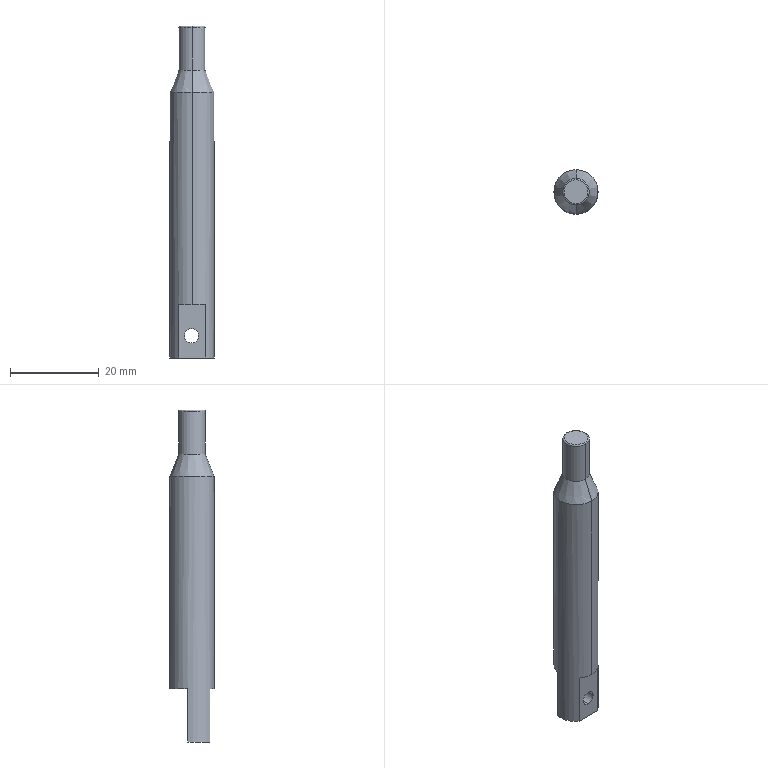Component | SolidWorks | CLS-MechanismOperatingAxisBracketAssembly.SLDPRT-1_CLS-MechanismPositioningPin-1 | 1 solid | 16 faces | box 10 x 10 x 75 mm | volume 4810 mm3 | cylinder 6 | plane 6 | torus 2 | cone 2 | commonest cylinder face diameters 3.2 x2 6 x2 10 x2
STEP:
#1=COLOUR_RGB('',0.7922,0.8196,0.9333);
#2=FILL_AREA_STYLE_COLOUR('',#1);
#3=FILL_AREA_STYLE('',(#2));
#4=SURFACE_STYLE_FILL_AREA(#3);
#5=SURFACE_SIDE_STYLE('',(#4));
#6=SURFACE_STYLE_USAGE(.BOTH.,#5);
#7=PRESENTATION_STYLE_ASSIGNMENT((#6));
#8=CARTESIAN_POINT('',(-2.328,-1.075,-2.122));
#9=VERTEX_POINT('',#8);
#10=CARTESIAN_POINT('',(-2.328,-1.075,-2.248));
#11=VERTEX_POINT('',#10);
#12=CARTESIAN_POINT('',(-2.328,-1.075,-2.185));
#13=DIRECTION('',(0.,-1.,0.));
#14=DIRECTION('',(0.,0.,-1.));
#15=AXIS2_PLACEMENT_3D('',#12,#13,#14);
#16=CIRCLE('',#15,0.06299);
#17=EDGE_CURVE('',#9,#11,#16,.T.);
#18=ORIENTED_EDGE('',*,*,#17,.T.);
#19=CARTESIAN_POINT('',(-2.328,-0.8783,-2.248));
#20=VERTEX_POINT('',#19);
#21=CARTESIAN_POINT('',(-2.328,-1.114,-2.248));
#22=DIRECTION('',(-0.,1.,-0.));
#23=VECTOR('',#22,39.37);
#24=LINE('',#21,#23);
#25=EDGE_CURVE('',#11,#20,#24,.T.);
#26=ORIENTED_EDGE('',*,*,#25,.T.);
#27=CARTESIAN_POINT('',(-2.328,-0.8783,-2.122));
#28=VERTEX_POINT('',#27);
#29=CARTESIAN_POINT('',(-2.328,-0.8783,-2.185));
#30=DIRECTION('',(-0.,1.,-0.));
#31=DIRECTION('',(0.,0.,1.));
#32=AXIS2_PLACEMENT_3D('',#29,#30,#31);
#33=CIRCLE('',#32,0.06299);
#34=EDGE_CURVE('',#20,#28,#33,.T.);
#35=ORIENTED_EDGE('',*,*,#34,.T.);
#36=CARTESIAN_POINT('',(-2.328,-1.114,-2.122));
#37=DIRECTION('',(-0.,1.,-0.));
#38=VECTOR('',#37,39.37);
#39=LINE('',#36,#38);
#40=EDGE_CURVE('',#9,#28,#39,.T.);
#41=ORIENTED_EDGE('',*,*,#40,.F.);
#42=EDGE_LOOP('',(#18,#26,#35,#41));
#43=FACE_OUTER_BOUND('',#42,.T.);
#44=CARTESIAN_POINT('',(-2.328,-1.114,-2.185));
#45=DIRECTION('',(-0.,1.,-0.));
#46=DIRECTION('',(0.,0.,1.));
#47=AXIS2_PLACEMENT_3D('',#44,#45,#46);
#48=CYLINDRICAL_SURFACE('',#47,0.06299);
#49=ADVANCED_FACE('',(#43),#48,.F.);
#50=CARTESIAN_POINT('',(-2.324,-0.7995,0.5594));
#51=VERTEX_POINT('',#50);
#52=CARTESIAN_POINT('',(-2.324,-1.036,0.5594));
#53=VERTEX_POINT('',#52);
#54=CARTESIAN_POINT('',(-2.324,-0.9176,0.5594));
#55=DIRECTION('',(-0.,-0.,-1.));
#56=DIRECTION('',(0.,-1.,0.));
#57=AXIS2_PLACEMENT_3D('',#54,#55,#56);
#58=CIRCLE('',#57,0.1181);
#59=EDGE_CURVE('',#51,#53,#58,.T.);
#60=ORIENTED_EDGE('',*,*,#59,.F.);
#61=CARTESIAN_POINT('',(-2.324,-0.8113,0.5712));
#62=VERTEX_POINT('',#61);
#63=CARTESIAN_POINT('',(-2.324,-0.8113,0.5594));
#64=DIRECTION('',(1.,-0.,-0.));
#65=DIRECTION('',(0.,1.,0.));
#66=AXIS2_PLACEMENT_3D('',#63,#64,#65);
#67=CIRCLE('',#66,0.01181);
#68=EDGE_CURVE('',#51,#62,#67,.T.);
#69=ORIENTED_EDGE('',*,*,#68,.T.);
#70=CARTESIAN_POINT('',(-2.324,-1.024,0.5712));
#71=VERTEX_POINT('',#70);
#72=CARTESIAN_POINT('',(-2.324,-0.9176,0.5712));
#73=DIRECTION('',(0.,0.,1.));
#74=DIRECTION('',(0.,-1.,0.));
#75=AXIS2_PLACEMENT_3D('',#72,#73,#74);
#76=CIRCLE('',#75,0.1063);
#77=EDGE_CURVE('',#71,#62,#76,.T.);
#78=ORIENTED_EDGE('',*,*,#77,.F.);
#79=CARTESIAN_POINT('',(-2.324,-1.024,0.5594));
#80=DIRECTION('',(-1.,-0.,0.));
#81=DIRECTION('',(0.,0.,1.));
#82=AXIS2_PLACEMENT_3D('',#79,#80,#81);
#83=CIRCLE('',#82,0.01181);
#84=EDGE_CURVE('',#53,#71,#83,.T.);
#85=ORIENTED_EDGE('',*,*,#84,.F.);
#86=EDGE_LOOP('',(#60,#69,#78,#85));
#87=FACE_OUTER_BOUND('',#86,.T.);
#88=CARTESIAN_POINT('',(-2.324,-0.9176,0.5594));
#89=DIRECTION('',(0.,0.,1.));
#90=DIRECTION('',(0.,-1.,0.));
#91=AXIS2_PLACEMENT_3D('',#88,#89,#90);
#92=TOROIDAL_SURFACE('',#91,0.1063,0.01181);
#93=ADVANCED_FACE('',(#87),#92,.T.);
#94=ORIENTED_EDGE('',*,*,#59,.T.);
#95=CARTESIAN_POINT('',(-2.324,-1.036,0.1775));
#96=VERTEX_POINT('',#95);
#97=CARTESIAN_POINT('',(-2.324,-1.036,0.5712));
#98=DIRECTION('',(-0.,-0.,-1.));
#99=VECTOR('',#98,39.37);
#100=LINE('',#97,#99);
#101=EDGE_CURVE('',#53,#96,#100,.T.);
#102=ORIENTED_EDGE('',*,*,#101,.T.);
#103=CARTESIAN_POINT('',(-2.324,-0.7995,0.1775));
#104=VERTEX_POINT('',#103);
#105=CARTESIAN_POINT('',(-2.324,-0.9176,0.1775));
#106=DIRECTION('',(0.,0.,1.));
#107=DIRECTION('',(0.,-1.,0.));
#108=AXIS2_PLACEMENT_3D('',#105,#106,#107);
#109=CIRCLE('',#108,0.1181);
#110=EDGE_CURVE('',#96,#104,#109,.T.);
#111=ORIENTED_EDGE('',*,*,#110,.T.);
#112=CARTESIAN_POINT('',(-2.324,-0.7995,0.5712));
#113=DIRECTION('',(-0.,-0.,-1.));
#114=VECTOR('',#113,39.37);
#115=LINE('',#112,#114);
#116=EDGE_CURVE('',#51,#104,#115,.T.);
#117=ORIENTED_EDGE('',*,*,#116,.F.);
#118=EDGE_LOOP('',(#94,#102,#111,#117));
#119=FACE_OUTER_BOUND('',#118,.T.);
#120=CARTESIAN_POINT('',(-2.324,-0.9176,0.5712));
#121=DIRECTION('',(-0.,-0.,-1.));
#122=DIRECTION('',(0.,1.,0.));
#123=AXIS2_PLACEMENT_3D('',#120,#121,#122);
#124=CYLINDRICAL_SURFACE('',#123,0.1181);
#125=ADVANCED_FACE('',(#119),#124,.T.);
#126=ORIENTED_EDGE('',*,*,#110,.F.);
#127=CARTESIAN_POINT('',(-2.324,-1.114,-0.01935));
#128=VERTEX_POINT('',#127);
#129=CARTESIAN_POINT('',(-2.324,-1.036,0.1775));
#130=DIRECTION('',(0.,-0.3714,-0.9285));
#131=VECTOR('',#130,39.37);
#132=LINE('',#129,#131);
#133=EDGE_CURVE('',#96,#128,#132,.T.);
#134=ORIENTED_EDGE('',*,*,#133,.T.);
#135=CARTESIAN_POINT('',(-2.324,-0.7208,-0.01935));
#136=VERTEX_POINT('',#135);
#137=CARTESIAN_POINT('',(-2.324,-0.9176,-0.01935));
#138=DIRECTION('',(-0.,-0.,-1.));
#139=DIRECTION('',(0.,-1.,0.));
#140=AXIS2_PLACEMENT_3D('',#137,#138,#139);
#141=CIRCLE('',#140,0.1969);
#142=EDGE_CURVE('',#136,#128,#141,.T.);
#143=ORIENTED_EDGE('',*,*,#142,.F.);
#144=CARTESIAN_POINT('',(-2.324,-0.7995,0.1775));
#145=DIRECTION('',(-0.,0.3714,-0.9285));
#146=VECTOR('',#145,39.37);
#147=LINE('',#144,#146);
#148=EDGE_CURVE('',#104,#136,#147,.T.);
#149=ORIENTED_EDGE('',*,*,#148,.F.);
#150=EDGE_LOOP('',(#126,#134,#143,#149));
#151=FACE_OUTER_BOUND('',#150,.T.);
#152=CARTESIAN_POINT('',(-2.324,-0.9176,0.1775));
#153=DIRECTION('',(-0.,-0.,-1.));
#154=DIRECTION('',(0.,1.,-0.));
#155=AXIS2_PLACEMENT_3D('',#152,#153,#154);
#156=CONICAL_SURFACE('',#155,0.1181,0.3805);
#157=ADVANCED_FACE('',(#151),#156,.T.);
#158=ORIENTED_EDGE('',*,*,#142,.T.);
#159=CARTESIAN_POINT('',(-2.324,-1.114,-1.909));
#160=VERTEX_POINT('',#159);
#161=CARTESIAN_POINT('',(-2.324,-1.114,0.1775));
#162=DIRECTION('',(-0.,-0.,-1.));
#163=VECTOR('',#162,39.37);
#164=LINE('',#161,#163);
#165=EDGE_CURVE('',#128,#160,#164,.T.);
#166=ORIENTED_EDGE('',*,*,#165,.T.);
#167=CARTESIAN_POINT('',(-2.206,-1.075,-1.909));
#168=VERTEX_POINT('',#167);
#169=CARTESIAN_POINT('',(-2.324,-0.9176,-1.909));
#170=DIRECTION('',(-0.,-0.,-1.));
#171=DIRECTION('',(0.,1.,0.));
#172=AXIS2_PLACEMENT_3D('',#169,#170,#171);
#173=CIRCLE('',#172,0.1969);
#174=EDGE_CURVE('',#168,#160,#173,.T.);
#175=ORIENTED_EDGE('',*,*,#174,.F.);
#176=CARTESIAN_POINT('',(-2.206,-1.075,-2.382));
#177=VERTEX_POINT('',#176);
#178=CARTESIAN_POINT('',(-2.206,-1.075,-1.909));
#179=DIRECTION('',(-0.,-0.,-1.));
#180=VECTOR('',#179,39.37);
#181=LINE('',#178,#180);
#182=EDGE_CURVE('',#168,#177,#181,.T.);
#183=ORIENTED_EDGE('',*,*,#182,.T.);
#184=CARTESIAN_POINT('',(-2.131,-0.8783,-2.382));
#185=VERTEX_POINT('',#184);
#186=CARTESIAN_POINT('',(-2.324,-0.9176,-2.382));
#187=DIRECTION('',(0.,0.,1.));
#188=DIRECTION('',(0.,-1.,0.));
#189=AXIS2_PLACEMENT_3D('',#186,#187,#188);
#190=CIRCLE('',#189,0.1969);
#191=EDGE_CURVE('',#177,#185,#190,.T.);
#192=ORIENTED_EDGE('',*,*,#191,.T.);
#193=CARTESIAN_POINT('',(-2.131,-0.8783,-1.909));
#194=VERTEX_POINT('',#193);
#195=CARTESIAN_POINT('',(-2.131,-0.8783,-1.909));
#196=DIRECTION('',(-0.,-0.,-1.));
#197=VECTOR('',#196,39.37);
#198=LINE('',#195,#197);
#199=EDGE_CURVE('',#194,#185,#198,.T.);
#200=ORIENTED_EDGE('',*,*,#199,.F.);
#201=CARTESIAN_POINT('',(-2.324,-0.7208,-1.909));
#202=VERTEX_POINT('',#201);
#203=CARTESIAN_POINT('',(-2.324,-0.9176,-1.909));
#204=DIRECTION('',(-0.,-0.,-1.));
#205=DIRECTION('',(0.,1.,0.));
#206=AXIS2_PLACEMENT_3D('',#203,#204,#205);
#207=CIRCLE('',#206,0.1969);
#208=EDGE_CURVE('',#202,#194,#207,.T.);
#209=ORIENTED_EDGE('',*,*,#208,.F.);
#210=CARTESIAN_POINT('',(-2.324,-0.7208,0.1775));
#211=DIRECTION('',(-0.,-0.,-1.));
#212=VECTOR('',#211,39.37);
#213=LINE('',#210,#212);
#214=EDGE_CURVE('',#136,#202,#213,.T.);
#215=ORIENTED_EDGE('',*,*,#214,.F.);
#216=EDGE_LOOP('',(#158,#166,#175,#183,#192,#200,#209,#215));
#217=FACE_OUTER_BOUND('',#216,.T.);
#218=CARTESIAN_POINT('',(-2.324,-0.9176,0.1775));
#219=DIRECTION('',(-0.,-0.,-1.));
#220=DIRECTION('',(0.,1.,-0.));
#221=AXIS2_PLACEMENT_3D('',#218,#219,#220);
#222=CYLINDRICAL_SURFACE('',#221,0.1969);
#223=ADVANCED_FACE('',(#217),#222,.T.);
#224=ORIENTED_EDGE('',*,*,#165,.F.);
#225=CARTESIAN_POINT('',(-2.324,-0.9176,-0.01935));
#226=DIRECTION('',(-0.,-0.,-1.));
#227=DIRECTION('',(0.,-1.,0.));
#228=AXIS2_PLACEMENT_3D('',#225,#226,#227);
#229=CIRCLE('',#228,0.1969);
#230=EDGE_CURVE('',#128,#136,#229,.T.);
#231=ORIENTED_EDGE('',*,*,#230,.T.);
#232=ORIENTED_EDGE('',*,*,#214,.T.);
#233=CARTESIAN_POINT('',(-2.517,-0.8783,-1.909));
#234=VERTEX_POINT('',#233);
#235=CARTESIAN_POINT('',(-2.324,-0.9176,-1.909));
#236=DIRECTION('',(-0.,-0.,-1.));
#237=DIRECTION('',(0.,1.,0.));
#238=AXIS2_PLACEMENT_3D('',#235,#236,#237);
#239=CIRCLE('',#238,0.1969);
#240=EDGE_CURVE('',#234,#202,#239,.T.);
#241=ORIENTED_EDGE('',*,*,#240,.F.);
#242=CARTESIAN_POINT('',(-2.517,-0.8783,-2.382));
#243=VERTEX_POINT('',#242);
#244=CARTESIAN_POINT('',(-2.517,-0.8783,-1.909));
#245=DIRECTION('',(-0.,-0.,-1.));
#246=VECTOR('',#245,39.37);
#247=LINE('',#244,#246);
#248=EDGE_CURVE('',#234,#243,#247,.T.);
#249=ORIENTED_EDGE('',*,*,#248,.T.);
#250=CARTESIAN_POINT('',(-2.442,-1.075,-2.382));
#251=VERTEX_POINT('',#250);
#252=CARTESIAN_POINT('',(-2.324,-0.9176,-2.382));
#253=DIRECTION('',(0.,0.,1.));
#254=DIRECTION('',(0.,-1.,0.));
#255=AXIS2_PLACEMENT_3D('',#252,#253,#254);
#256=CIRCLE('',#255,0.1969);
#257=EDGE_CURVE('',#243,#251,#256,.T.);
#258=ORIENTED_EDGE('',*,*,#257,.T.);
#259=CARTESIAN_POINT('',(-2.442,-1.075,-1.909));
#260=VERTEX_POINT('',#259);
#261=CARTESIAN_POINT('',(-2.442,-1.075,-1.909));
#262=DIRECTION('',(-0.,-0.,-1.));
#263=VECTOR('',#262,39.37);
#264=LINE('',#261,#263);
#265=EDGE_CURVE('',#260,#251,#264,.T.);
#266=ORIENTED_EDGE('',*,*,#265,.F.);
#267=CARTESIAN_POINT('',(-2.324,-0.9176,-1.909));
#268=DIRECTION('',(-0.,-0.,-1.));
#269=DIRECTION('',(0.,1.,0.));
#270=AXIS2_PLACEMENT_3D('',#267,#268,#269);
#271=CIRCLE('',#270,0.1969);
#272=EDGE_CURVE('',#160,#260,#271,.T.);
#273=ORIENTED_EDGE('',*,*,#272,.F.);
#274=EDGE_LOOP('',(#224,#231,#232,#241,#249,#258,#266,#273));
#275=FACE_OUTER_BOUND('',#274,.T.);
#276=CARTESIAN_POINT('',(-2.324,-0.9176,0.1775));
#277=DIRECTION('',(-0.,-0.,-1.));
#278=DIRECTION('',(0.,1.,-0.));
#279=AXIS2_PLACEMENT_3D('',#276,#277,#278);
#280=CYLINDRICAL_SURFACE('',#279,0.1969);
#281=ADVANCED_FACE('',(#275),#280,.T.);
#282=CARTESIAN_POINT('',(-2.324,-1.075,-2.382));
#283=DIRECTION('',(-1.,-0.,0.));
#284=VECTOR('',#283,39.37);
#285=LINE('',#282,#284);
#286=EDGE_CURVE('',#177,#251,#285,.T.);
#287=ORIENTED_EDGE('',*,*,#286,.T.);
#288=ORIENTED_EDGE('',*,*,#257,.F.);
#289=CARTESIAN_POINT('',(-2.324,-0.8783,-2.382));
#290=DIRECTION('',(1.,0.,-0.));
#291=VECTOR('',#290,39.37);
#292=LINE('',#289,#291);
#293=EDGE_CURVE('',#243,#185,#292,.T.);
#294=ORIENTED_EDGE('',*,*,#293,.T.);
#295=ORIENTED_EDGE('',*,*,#191,.F.);
#296=EDGE_LOOP('',(#287,#288,#294,#295));
#297=FACE_OUTER_BOUND('',#296,.T.);
#298=CARTESIAN_POINT('',(-2.324,-0.9176,-2.382));
#299=DIRECTION('',(0.,0.,1.));
#300=DIRECTION('',(0.,-1.,0.));
#301=AXIS2_PLACEMENT_3D('',#298,#299,#300);
#302=PLANE('',#301);
#303=ADVANCED_FACE('',(#297),#302,.F.);
#304=ORIENTED_EDGE('',*,*,#133,.F.);
#305=CARTESIAN_POINT('',(-2.324,-0.9176,0.1775));
#306=DIRECTION('',(0.,0.,1.));
#307=DIRECTION('',(0.,-1.,0.));
#308=AXIS2_PLACEMENT_3D('',#305,#306,#307);
#309=CIRCLE('',#308,0.1181);
#310=EDGE_CURVE('',#104,#96,#309,.T.);
#311=ORIENTED_EDGE('',*,*,#310,.F.);
#312=ORIENTED_EDGE('',*,*,#148,.T.);
#313=ORIENTED_EDGE('',*,*,#230,.F.);
#314=EDGE_LOOP('',(#304,#311,#312,#313));
#315=FACE_OUTER_BOUND('',#314,.T.);
#316=CARTESIAN_POINT('',(-2.324,-0.9176,0.1775));
#317=DIRECTION('',(-0.,-0.,-1.));
#318=DIRECTION('',(0.,1.,-0.));
#319=AXIS2_PLACEMENT_3D('',#316,#317,#318);
#320=CONICAL_SURFACE('',#319,0.1181,0.3805);
#321=ADVANCED_FACE('',(#315),#320,.T.);
#322=ORIENTED_EDGE('',*,*,#101,.F.);
#323=CARTESIAN_POINT('',(-2.324,-0.9176,0.5594));
#324=DIRECTION('',(-0.,-0.,-1.));
#325=DIRECTION('',(0.,-1.,0.));
#326=AXIS2_PLACEMENT_3D('',#323,#324,#325);
#327=CIRCLE('',#326,0.1181);
#328=EDGE_CURVE('',#53,#51,#327,.T.);
#329=ORIENTED_EDGE('',*,*,#328,.T.);
#330=ORIENTED_EDGE('',*,*,#116,.T.);
#331=ORIENTED_EDGE('',*,*,#310,.T.);
#332=EDGE_LOOP('',(#322,#329,#330,#331));
#333=FACE_OUTER_BOUND('',#332,.T.);
#334=CARTESIAN_POINT('',(-2.324,-0.9176,0.5712));
#335=DIRECTION('',(-0.,-0.,-1.));
#336=DIRECTION('',(0.,1.,0.));
#337=AXIS2_PLACEMENT_3D('',#334,#335,#336);
#338=CYLINDRICAL_SURFACE('',#337,0.1181);
#339=ADVANCED_FACE('',(#333),#338,.T.);
#340=ORIENTED_EDGE('',*,*,#77,.T.);
#341=CARTESIAN_POINT('',(-2.324,-0.9176,0.5712));
#342=DIRECTION('',(0.,0.,1.));
#343=DIRECTION('',(0.,-1.,0.));
#344=AXIS2_PLACEMENT_3D('',#341,#342,#343);
#345=CIRCLE('',#344,0.1063);
#346=EDGE_CURVE('',#62,#71,#345,.T.);
#347=ORIENTED_EDGE('',*,*,#346,.T.);
#348=EDGE_LOOP('',(#340,#347));
#349=FACE_OUTER_BOUND('',#348,.T.);
#350=CARTESIAN_POINT('',(-2.324,-0.9176,0.5712));
#351=DIRECTION('',(0.,0.,1.));
#352=DIRECTION('',(0.,-1.,0.));
#353=AXIS2_PLACEMENT_3D('',#350,#351,#352);
#354=PLANE('',#353);
#355=ADVANCED_FACE('',(#349),#354,.T.);
#356=ORIENTED_EDGE('',*,*,#68,.F.);
#357=ORIENTED_EDGE('',*,*,#328,.F.);
#358=ORIENTED_EDGE('',*,*,#84,.T.);
#359=ORIENTED_EDGE('',*,*,#346,.F.);
#360=EDGE_LOOP('',(#356,#357,#358,#359));
#361=FACE_OUTER_BOUND('',#360,.T.);
#362=CARTESIAN_POINT('',(-2.324,-0.9176,0.5594));
#363=DIRECTION('',(0.,0.,1.));
#364=DIRECTION('',(0.,-1.,0.));
#365=AXIS2_PLACEMENT_3D('',#362,#363,#364);
#366=TOROIDAL_SURFACE('',#365,0.1063,0.01181);
#367=ADVANCED_FACE('',(#361),#366,.T.);
#368=CARTESIAN_POINT('',(-2.328,-0.8783,-2.185));
#369=DIRECTION('',(-0.,1.,-0.));
#370=DIRECTION('',(0.,0.,1.));
#371=AXIS2_PLACEMENT_3D('',#368,#369,#370);
#372=CIRCLE('',#371,0.06299);
#373=EDGE_CURVE('',#28,#20,#372,.T.);
#374=ORIENTED_EDGE('',*,*,#373,.F.);
#375=ORIENTED_EDGE('',*,*,#34,.F.);
#376=EDGE_LOOP('',(#374,#375));
#377=FACE_BOUND('',#376,.T.);
#378=ORIENTED_EDGE('',*,*,#293,.F.);
#379=ORIENTED_EDGE('',*,*,#248,.F.);
#380=CARTESIAN_POINT('',(-2.324,-0.8783,-1.909));
#381=DIRECTION('',(1.,0.,-0.));
#382=VECTOR('',#381,39.37);
#383=LINE('',#380,#382);
#384=EDGE_CURVE('',#234,#194,#383,.T.);
#385=ORIENTED_EDGE('',*,*,#384,.T.);
#386=ORIENTED_EDGE('',*,*,#199,.T.);
#387=EDGE_LOOP('',(#378,#379,#385,#386));
#388=FACE_OUTER_BOUND('',#387,.T.);
#389=CARTESIAN_POINT('',(-2.324,-0.8783,-1.909));
#390=DIRECTION('',(-0.,1.,-0.));
#391=DIRECTION('',(0.,0.,1.));
#392=AXIS2_PLACEMENT_3D('',#389,#390,#391);
#393=PLANE('',#392);
#394=ADVANCED_FACE('',(#377,#388),#393,.T.);
#395=ORIENTED_EDGE('',*,*,#384,.F.);
#396=ORIENTED_EDGE('',*,*,#240,.T.);
#397=ORIENTED_EDGE('',*,*,#208,.T.);
#398=EDGE_LOOP('',(#395,#396,#397));
#399=FACE_OUTER_BOUND('',#398,.T.);
#400=CARTESIAN_POINT('',(-2.324,-0.9176,-1.909));
#401=DIRECTION('',(-0.,-0.,-1.));
#402=DIRECTION('',(-0.,1.,-0.));
#403=AXIS2_PLACEMENT_3D('',#400,#401,#402);
#404=PLANE('',#403);
#405=ADVANCED_FACE('',(#399),#404,.T.);
#406=ORIENTED_EDGE('',*,*,#17,.F.);
#407=CARTESIAN_POINT('',(-2.328,-1.075,-2.185));
#408=DIRECTION('',(0.,-1.,0.));
#409=DIRECTION('',(0.,0.,-1.));
#410=AXIS2_PLACEMENT_3D('',#407,#408,#409);
#411=CIRCLE('',#410,0.06299);
#412=EDGE_CURVE('',#11,#9,#411,.T.);
#413=ORIENTED_EDGE('',*,*,#412,.F.);
#414=EDGE_LOOP('',(#406,#413));
#415=FACE_BOUND('',#414,.T.);
#416=ORIENTED_EDGE('',*,*,#286,.F.);
#417=ORIENTED_EDGE('',*,*,#182,.F.);
#418=CARTESIAN_POINT('',(-2.324,-1.075,-1.909));
#419=DIRECTION('',(-1.,-0.,0.));
#420=VECTOR('',#419,39.37);
#421=LINE('',#418,#420);
#422=EDGE_CURVE('',#168,#260,#421,.T.);
#423=ORIENTED_EDGE('',*,*,#422,.T.);
#424=ORIENTED_EDGE('',*,*,#265,.T.);
#425=EDGE_LOOP('',(#416,#417,#423,#424));
#426=FACE_OUTER_BOUND('',#425,.T.);
#427=CARTESIAN_POINT('',(-2.324,-1.075,-1.909));
#428=DIRECTION('',(0.,-1.,0.));
#429=DIRECTION('',(-0.,-0.,-1.));
#430=AXIS2_PLACEMENT_3D('',#427,#428,#429);
#431=PLANE('',#430);
#432=ADVANCED_FACE('',(#415,#426),#431,.T.);
#433=ORIENTED_EDGE('',*,*,#422,.F.);
#434=ORIENTED_EDGE('',*,*,#174,.T.);
#435=ORIENTED_EDGE('',*,*,#272,.T.);
#436=EDGE_LOOP('',(#433,#434,#435));
#437=FACE_OUTER_BOUND('',#436,.T.);
#438=CARTESIAN_POINT('',(-2.324,-0.9176,-1.909));
#439=DIRECTION('',(-0.,-0.,-1.));
#440=DIRECTION('',(-0.,1.,-0.));
#441=AXIS2_PLACEMENT_3D('',#438,#439,#440);
#442=PLANE('',#441);
#443=ADVANCED_FACE('',(#437),#442,.T.);
#444=ORIENTED_EDGE('',*,*,#25,.F.);
#445=ORIENTED_EDGE('',*,*,#412,.T.);
#446=ORIENTED_EDGE('',*,*,#40,.T.);
#447=ORIENTED_EDGE('',*,*,#373,.T.);
#448=EDGE_LOOP('',(#444,#445,#446,#447));
#449=FACE_OUTER_BOUND('',#448,.T.);
#450=CARTESIAN_POINT('',(-2.328,-1.114,-2.185));
#451=DIRECTION('',(-0.,1.,-0.));
#452=DIRECTION('',(0.,0.,1.));
#453=AXIS2_PLACEMENT_3D('',#450,#451,#452);
#454=CYLINDRICAL_SURFACE('',#453,0.06299);
#455=ADVANCED_FACE('',(#449),#454,.F.);
#456=CLOSED_SHELL('',(#49,#93,#125,#157,#223,#281,#303,#321,#339,#355,#367,#394,#405,#432,#443,#455));
#457=MANIFOLD_SOLID_BREP('',#456);
#458=STYLED_ITEM('',(#7),#457);
#459=(LENGTH_UNIT()NAMED_UNIT(*)SI_UNIT($,.METRE.));
#460=LENGTH_MEASURE_WITH_UNIT(LENGTH_MEASURE(0.0254),#459);
#461=DIMENSIONAL_EXPONENTS(1.,0.,0.,0.,0.,0.,0.);
#462=(CONVERSION_BASED_UNIT('',#460)LENGTH_UNIT()NAMED_UNIT(#461));
#463=UNCERTAINTY_MEASURE_WITH_UNIT(LENGTH_MEASURE(0.00001),#462,'','');
#464=(NAMED_UNIT(*)PLANE_ANGLE_UNIT()SI_UNIT($,.RADIAN.));
#465=(NAMED_UNIT(*)SI_UNIT($,.STERADIAN.)SOLID_ANGLE_UNIT());
#466=(GEOMETRIC_REPRESENTATION_CONTEXT(3)GLOBAL_UNCERTAINTY_ASSIGNED_CONTEXT((#463))GLOBAL_UNIT_ASSIGNED_CONTEXT((#462,#464,#465))REPRESENTATION_CONTEXT('',''));
#467=MECHANICAL_DESIGN_GEOMETRIC_PRESENTATION_REPRESENTATION('',(#458),#466);
#468=PRESENTATION_LAYER_ASSIGNMENT('','',(#458));
#469=CARTESIAN_POINT('',(0.,0.,0.));
#470=DIRECTION('',(0.,0.,1.));
#471=DIRECTION('',(1.,0.,0.));
#472=AXIS2_PLACEMENT_3D('',#469,#470,#471);
#473=(LENGTH_UNIT()NAMED_UNIT(*)SI_UNIT($,.METRE.));
#474=LENGTH_MEASURE_WITH_UNIT(LENGTH_MEASURE(0.0254),#473);
#475=DIMENSIONAL_EXPONENTS(1.,0.,0.,0.,0.,0.,0.);
#476=(CONVERSION_BASED_UNIT('',#474)LENGTH_UNIT()NAMED_UNIT(#475));
#477=UNCERTAINTY_MEASURE_WITH_UNIT(LENGTH_MEASURE(0.00001),#476,'','');
#478=(NAMED_UNIT(*)PLANE_ANGLE_UNIT()SI_UNIT($,.RADIAN.));
#479=(NAMED_UNIT(*)SI_UNIT($,.STERADIAN.)SOLID_ANGLE_UNIT());
#480=(GEOMETRIC_REPRESENTATION_CONTEXT(3)GLOBAL_UNCERTAINTY_ASSIGNED_CONTEXT((#477))GLOBAL_UNIT_ASSIGNED_CONTEXT((#476,#478,#479))REPRESENTATION_CONTEXT('',''));
#481=ADVANCED_BREP_SHAPE_REPRESENTATION('',(#457,#472),#480);